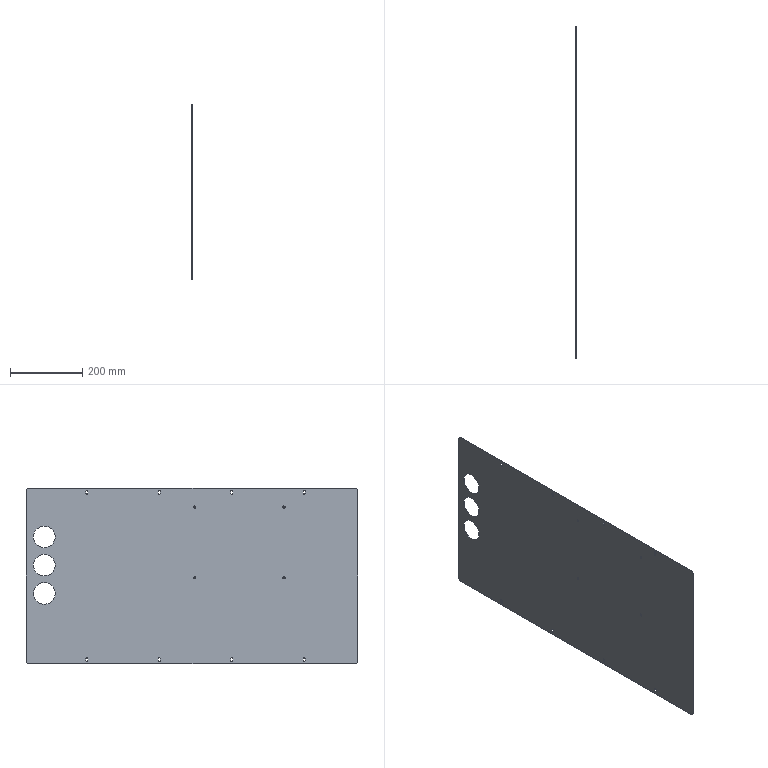Component | SolidWorks | MeteringChamberPartition400AType40001100-2 | 1 solid | 64 faces | volume 654127 mm3 | cylinder 42 | plane 22 | commonest cylinder face diameters 5.5 x24 6 x8 60 x6 20 x4